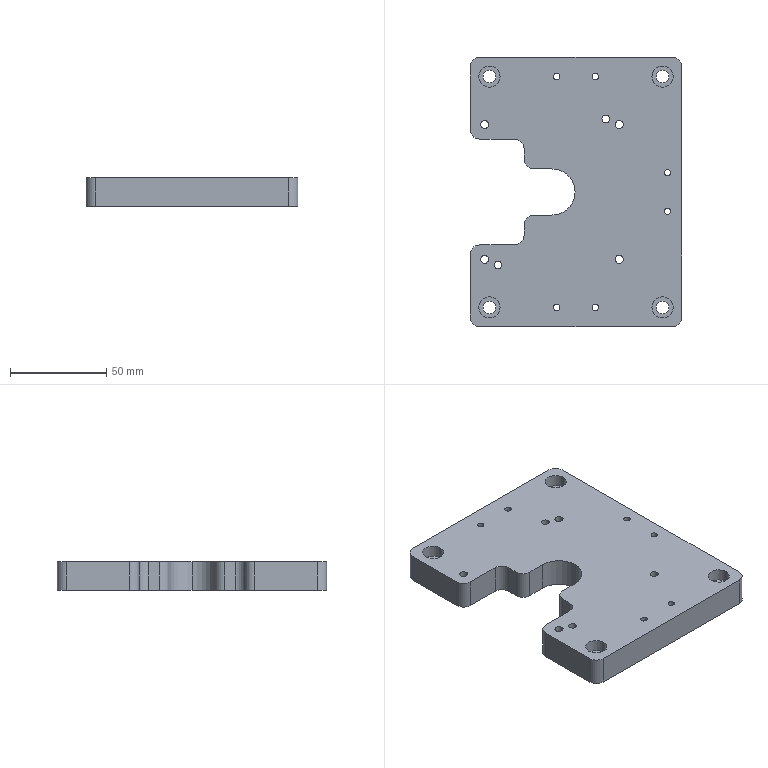Part | SolidWorks | mm | 1 solid | 81 faces | box 110 x 140 x 15 mm | volume 192076 mm3 | cylinder 60 | plane 21 | commonest cylinder face diameters 3.3 x12 10 x10 15 x8 4.2 x8 11 x8 6.6 x8 4 x4 24 x2
build123d program:
from build123d import *

# Parameters (mm, degrees)
SKETCH1_W                                       = 110
SKETCH1_H                                       = 140
BOSS_EXTRUDE1_DEPTH                             = 15
M6_HEX_SOCKET_HEAD_CAP_SCREW_CBORE1_D           = 6.6
M6_HEX_SOCKET_HEAD_CAP_SCREW_CBORE1_CBORE_D     = 11
M6_HEX_SOCKET_HEAD_CAP_SCREW_CBORE1_CBORE_DEPTH = 6.4
CUT_EXTRUDE1_DEPTH                              = 132.244
M5_TAPPED_HOLE1_D                               = 4.2
SIZE_MM_DOWEL_PIN_HOLE1_D                       = 4
SKETCH9_R                                       = 7.5
CUT_EXTRUDE2_DEPTH                              = 2
M4_TAPPED_HOLE1_D                               = 3.3
FILLET1_R                                       = 5


with BuildPart() as part:
    # Sketch1 → Boss-Extrude1 (new body)
    with BuildSketch(Plane.XY):
        with Locations((55, 0)):
            Rectangle(SKETCH1_W, SKETCH1_H)
    extrude(amount=BOSS_EXTRUDE1_DEPTH)

    # M6 Hex Socket Head Cap Screw CBORE1 (through all)
    with Locations(Plane.XY.offset(15)):
        with Locations((100, 60), (100, -60), (10, -60), (10, 60)):
            CounterBoreHole(M6_HEX_SOCKET_HEAD_CAP_SCREW_CBORE1_D / 2, M6_HEX_SOCKET_HEAD_CAP_SCREW_CBORE1_CBORE_D / 2, M6_HEX_SOCKET_HEAD_CAP_SCREW_CBORE1_CBORE_DEPTH)

    # Sketch4 → Cut-Extrude1 (cut, through all)
    with BuildSketch(Plane.XY.offset(15)):
        with BuildLine():
            Line((0, 27.5), (28, 27.5))
            Line((28, 27.5), (28, 12))
            Line((28, 12), (42.5, 12))
            ThreePointArc((42.5, 12), (54.5, 0), (42.5, -12))
            Line((42.5, -12), (28, -12))
            Line((28, -12), (28, -27.5))
            Line((28, -27.5), (0, -27.5))
            Line((0, -27.5), (0, 27.5))
        make_face()
    extrude(amount=-CUT_EXTRUDE1_DEPTH, mode=Mode.SUBTRACT)

    # M5 Tapped Hole1 (through all)
    with Locations(Plane.XY.offset(15)):
        with Locations((7.5, 35), (77.5, 35), (77.5, -35), (7.5, -35)):
            Hole(M5_TAPPED_HOLE1_D / 2)

    # Size mm Dowel Pin Hole1 (through all)
    with Locations(Plane.XY.offset(15)):
        with Locations((14.5, -38), (70.5, 38)):
            Hole(SIZE_MM_DOWEL_PIN_HOLE1_D / 2)

    # Sketch9 → Cut-Extrude2 (cut)
    with BuildSketch(Plane(origin=(0, 0, 0), x_dir=(-1, 0, 0), z_dir=(0, 0, -1))):
        with Locations((-100, 60)):
            Circle(SKETCH9_R)
        with Locations((-10, 60)):
            Circle(SKETCH9_R)
        with Locations((-100, -60)):
            Circle(SKETCH9_R)
        with Locations((-10, -60)):
            Circle(SKETCH9_R)
    extrude(amount=-CUT_EXTRUDE2_DEPTH, mode=Mode.SUBTRACT)

    # M4 Tapped Hole1 (through all)
    with Locations(Plane.XY.offset(15)):
        with Locations((102.5, 10), (102.5, -10), (65, 60), (45, 60), (45, -60), (65, -60)):
            Hole(M4_TAPPED_HOLE1_D / 2)

    # Fillet1
    fillet1_edges = [part.edges().sort_by_distance(p)[0] for p in [
        (0, -27.5, 7.5),
        (0, 27.5, 7.5),
        (28, 27.5, 7.5),
        (28, 12, 7.5),
        (28, -12, 7.5),
        (28, -27.5, 7.5),
        (0, 70, 7.5),
        (110, 70, 7.5),
        (110, -70, 7.5),
        (0, -70, 7.5),
    ]]
    fillet(fillet1_edges, radius=FILLET1_R)


solid = part.part